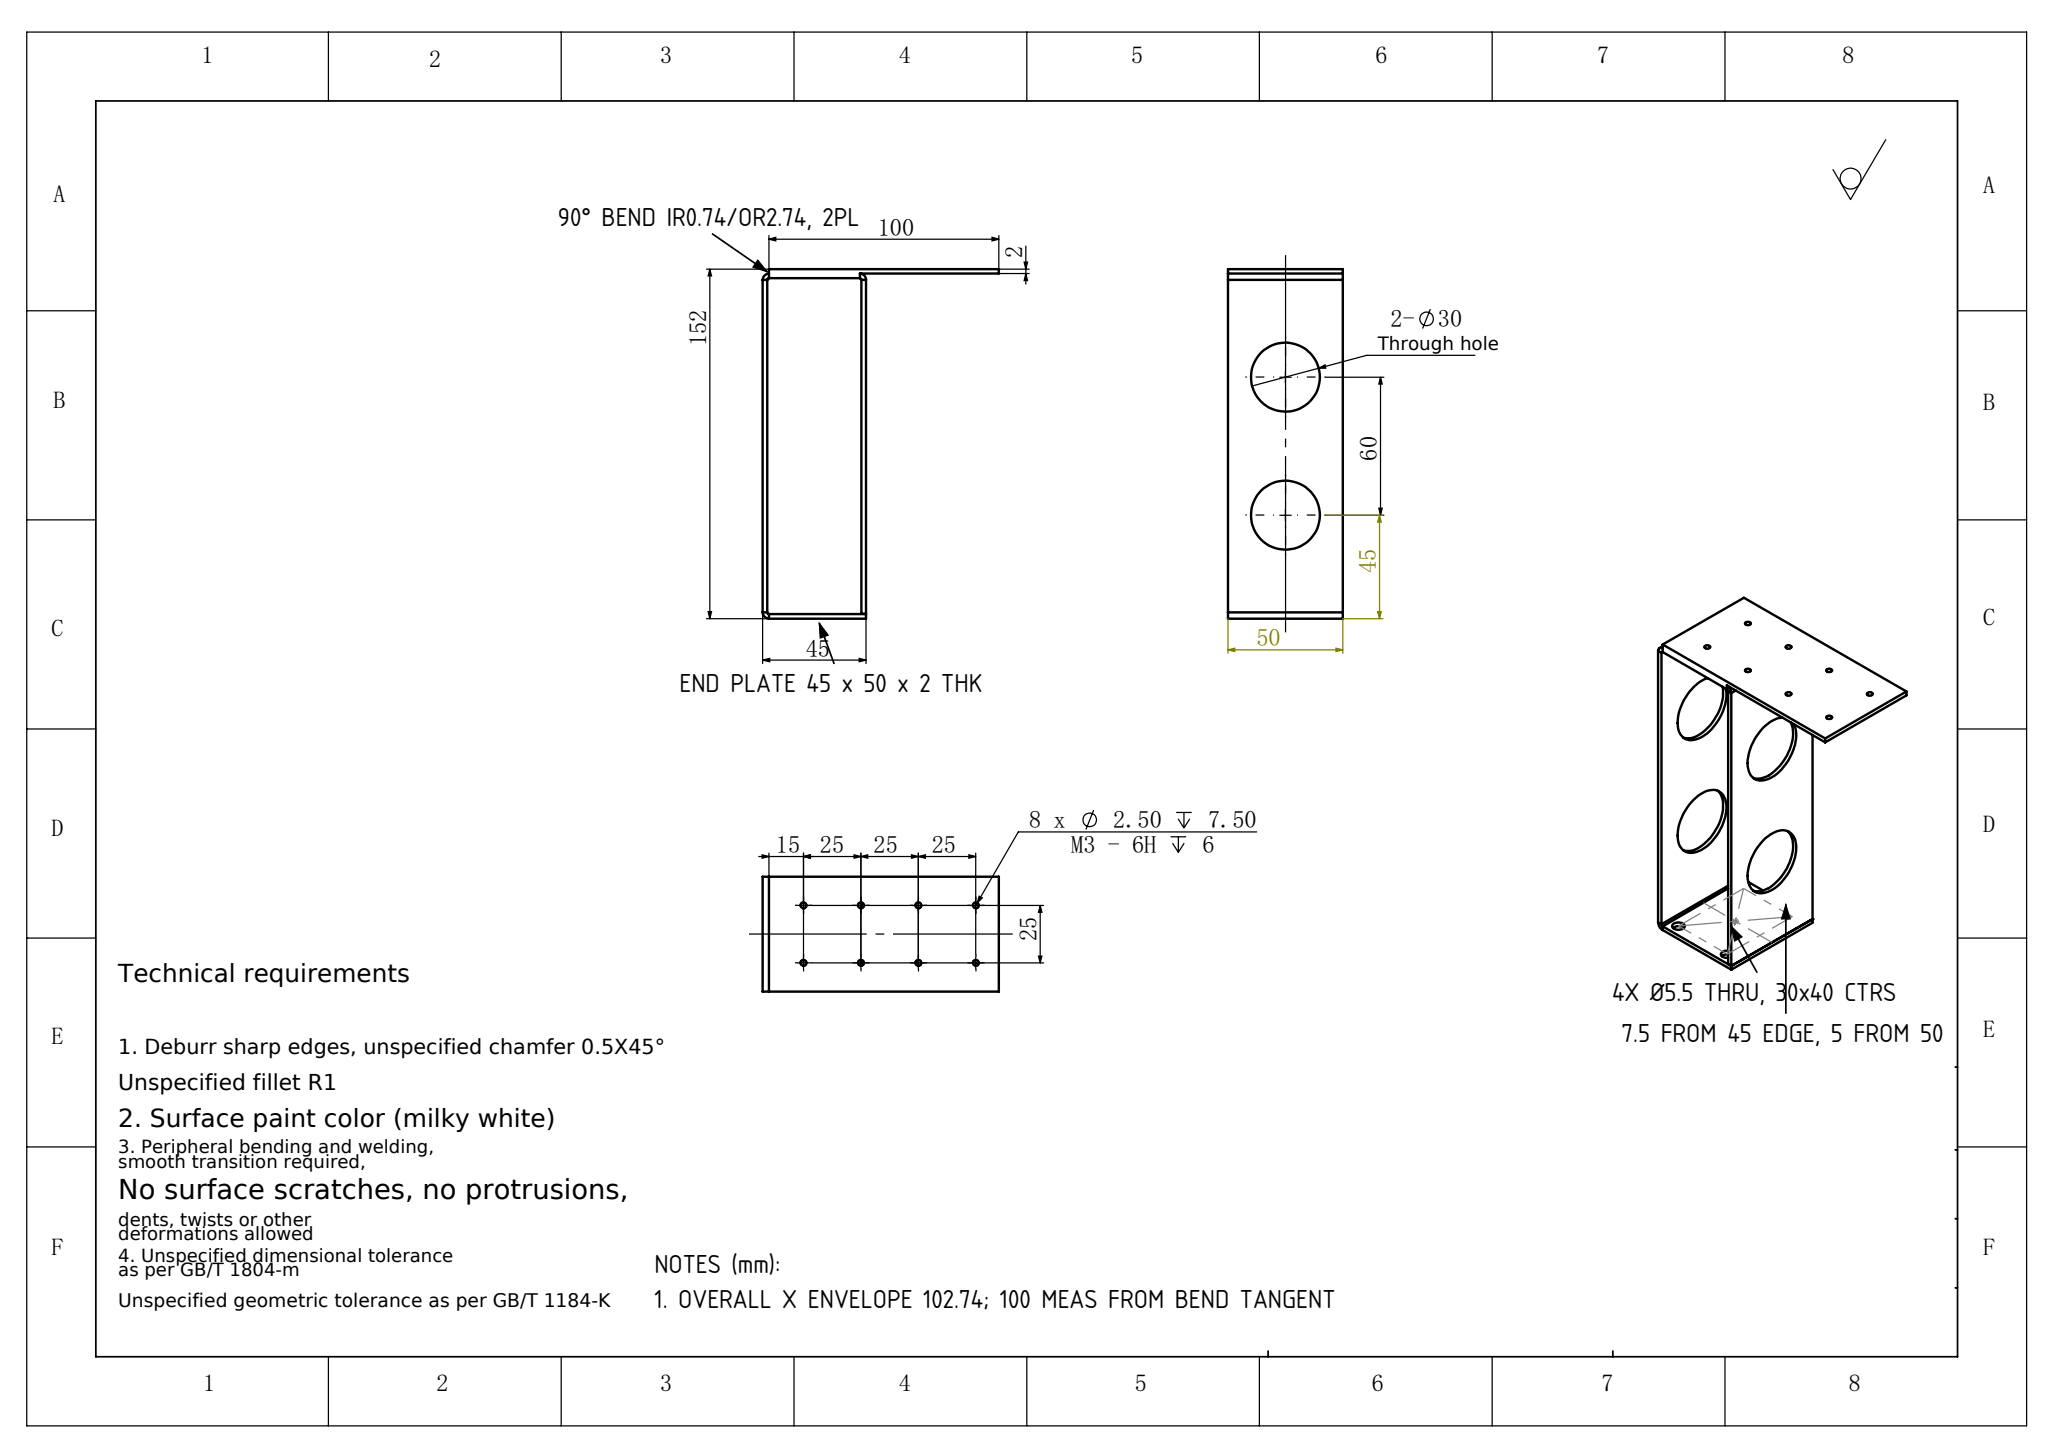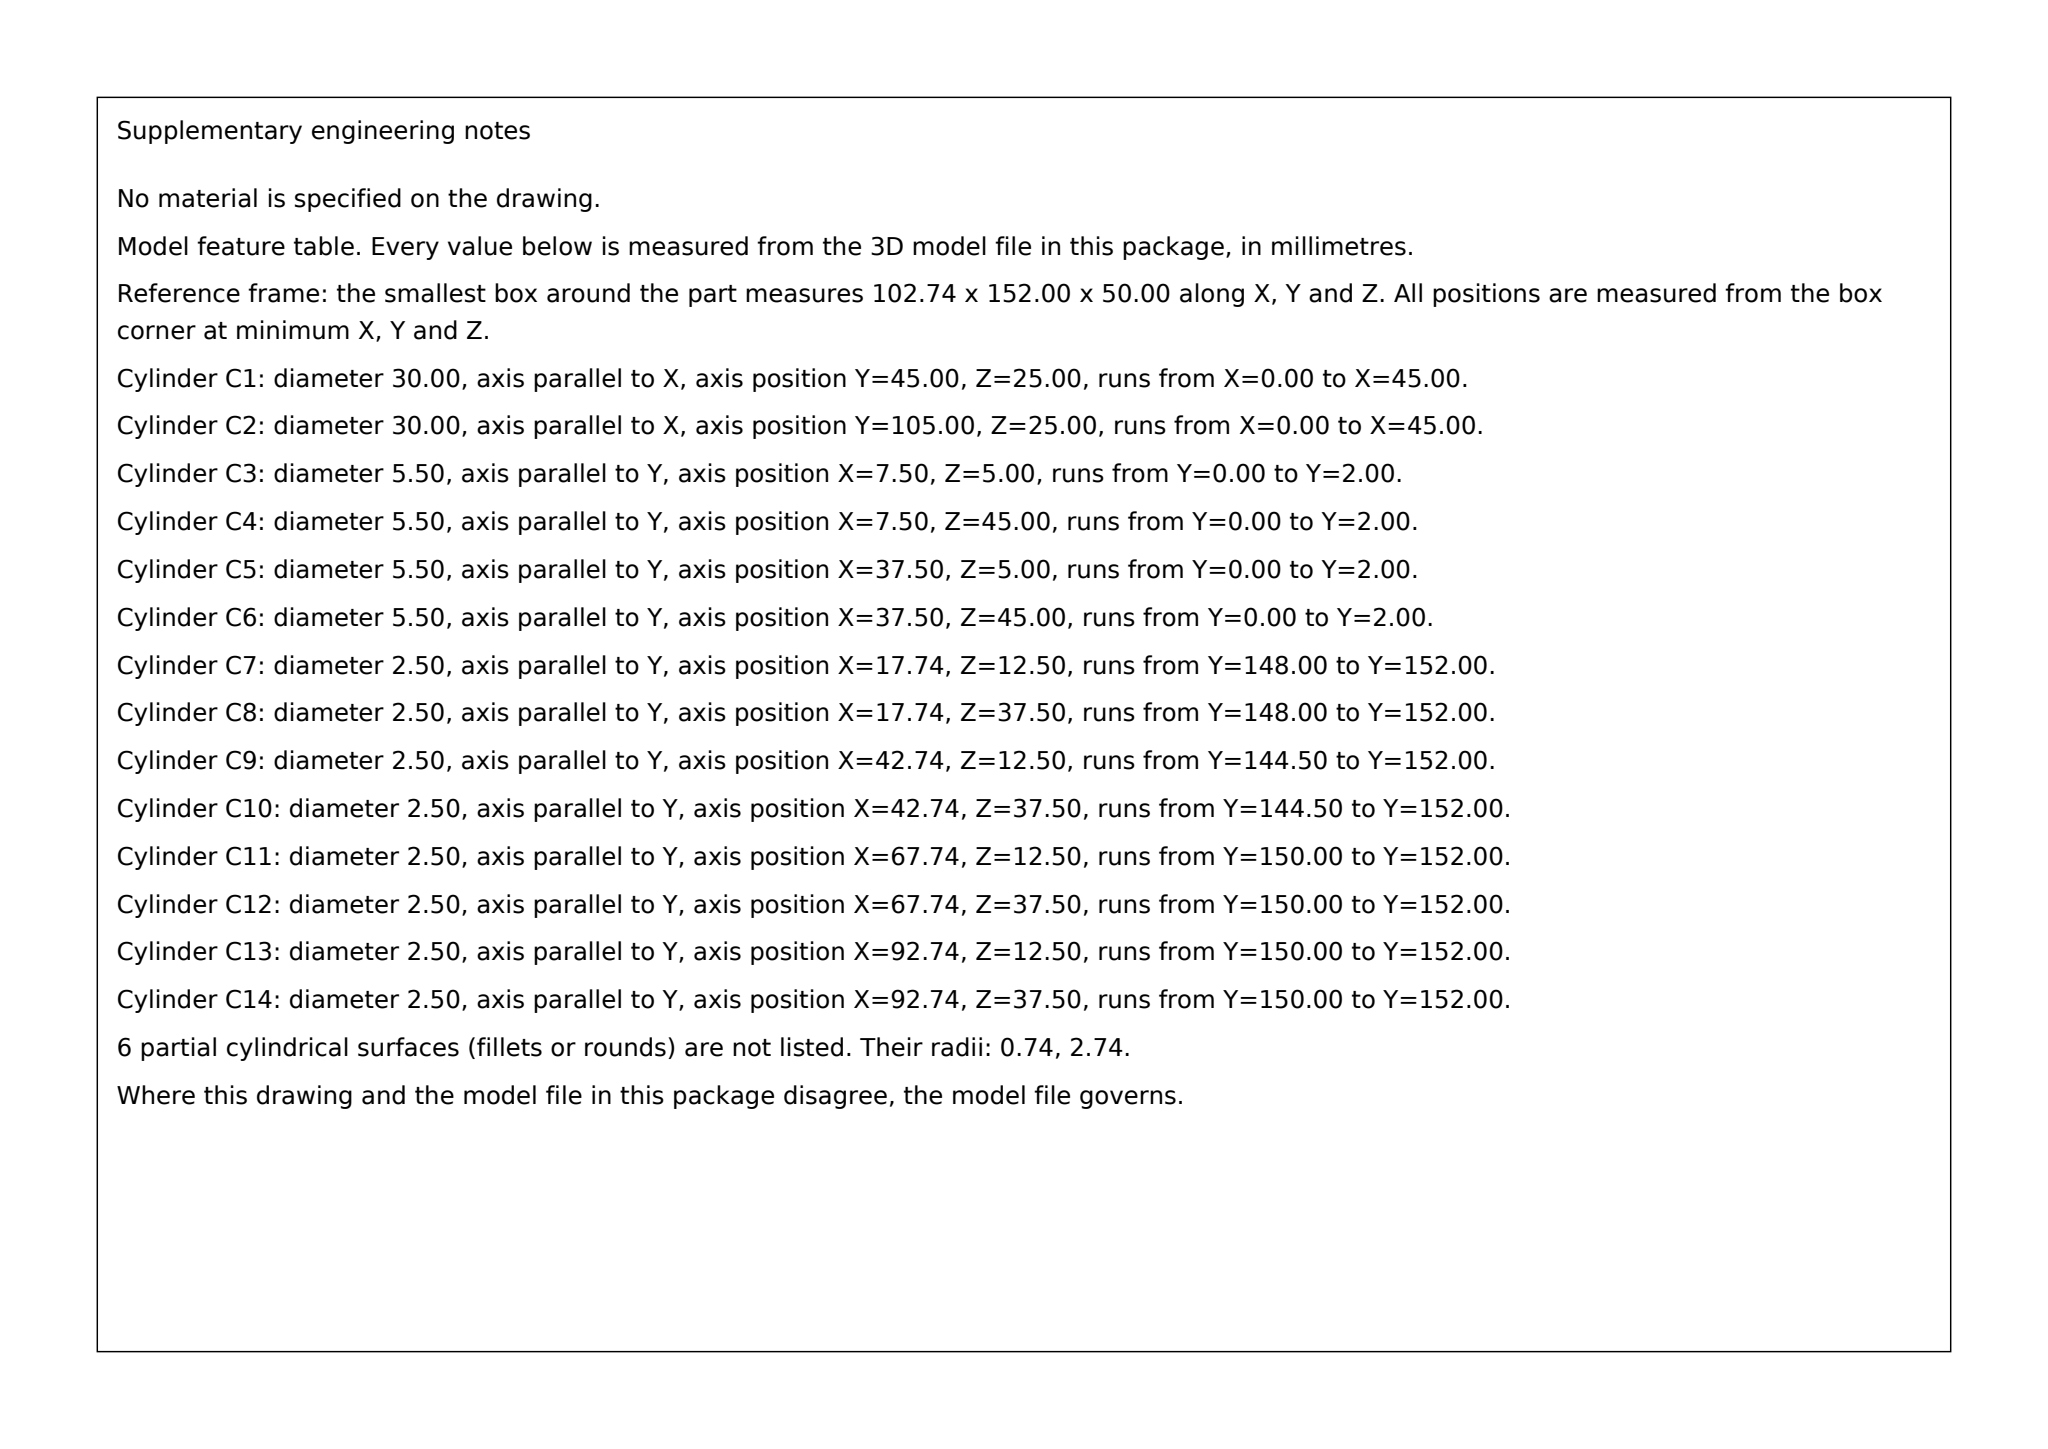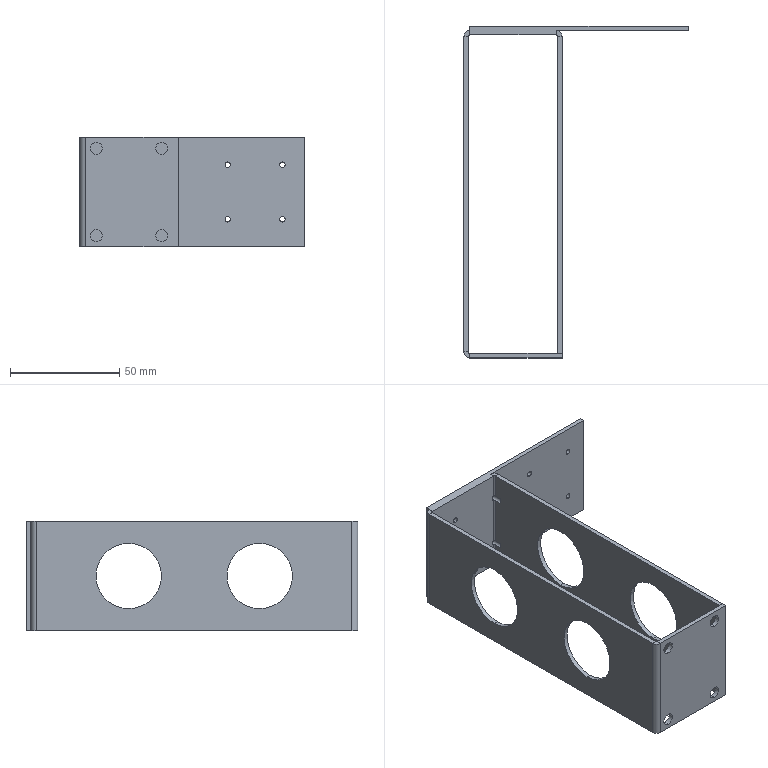Part | SolidWorks | mm | 1 solid | 71 faces | box 102.74 x 152 x 50 mm | volume 41996 mm3 | cylinder 42 | plane 27 | cone 2 | commonest cylinder face diameters 2.5 x18 30 x8 5.5 x8 1.473 x5 5.473 x3
Drawing notes:
BOTTOM PLATE: 4 x Ø5.5 THRU, 30 x 40 CTRS, CTD ON PLATE | from the solid: cyl dia 5.5 axis y len 2.0 at x=7.5/37.5, z=5/45; plate 45x50, ctr 22.5/25
BOTTOM PLATE 45 x 50 x 2 THK CLOSES OPEN END OF CHANNEL | from the solid: y-planes 0.0 and 2.0; x extent 0-45, z extent 0-50
2 PL 90° BEND: INSIDE R0.74, OUTSIDE R2.74 (R1 NOT APPLIC) | from the solid: cyl dia 1.473 (R0.74) and 5.473 (R2.74) axis z, len 50
OVERALL X ENVELOPE 102.74; 100 MEAS FROM BEND TANGENT | from the solid: bbox_xyz x=102.737; x-planes 2.74 and 102.74
4X Ø5.5 THRU: 7.5 FROM 45 EDGES, 5 FROM 50 EDGES (30X40 CTRS) | from the solid: 5.5 dia y-axis holes at x=7.5/37.5, z=5/45; plate 45 (x) x 50 (z), thk 2